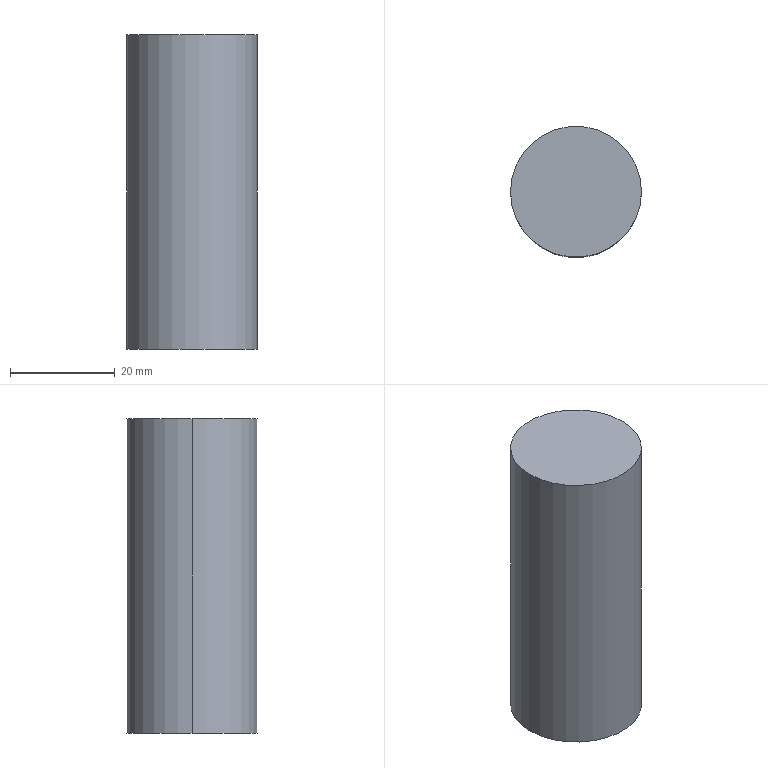Component | SolidWorks | Axis-1 | 1 solid | 4 faces | box 25 x 25 x 60 mm | volume 29452 mm3 | cylinder 2 | plane 2 | commonest cylinder face diameters 25 x2
build123d program:
from build123d import *

# Parameters (mm, degrees)
SKETCH1_R           = 12.5
BOSS_EXTRUDE1_DEPTH = 60


with BuildPart() as part:
    # Sketch1 → Boss-Extrude1 (new body)
    with BuildSketch(Plane.XY):
        Circle(SKETCH1_R)
    extrude(amount=BOSS_EXTRUDE1_DEPTH)


solid = part.part

# Placed as in the assembly
solid = solid.moved(Location((54.344, 1102.787, -13), (0, 0, 0)))
STEP:
#1=COLOUR_RGB('',0.7922,0.8196,0.9333);
#2=FILL_AREA_STYLE_COLOUR('',#1);
#3=FILL_AREA_STYLE('',(#2));
#4=SURFACE_STYLE_FILL_AREA(#3);
#5=SURFACE_SIDE_STYLE('',(#4));
#6=SURFACE_STYLE_USAGE(.BOTH.,#5);
#7=PRESENTATION_STYLE_ASSIGNMENT((#6));
#8=CARTESIAN_POINT('',(2.632,43.417,1.85));
#9=VERTEX_POINT('',#8);
#10=CARTESIAN_POINT('',(1.647,43.417,1.85));
#11=VERTEX_POINT('',#10);
#12=CARTESIAN_POINT('',(2.14,43.417,1.85));
#13=DIRECTION('',(0.,0.,1.));
#14=DIRECTION('',(1.,0.,0.));
#15=AXIS2_PLACEMENT_3D('',#12,#13,#14);
#16=CIRCLE('',#15,0.4921);
#17=EDGE_CURVE('',#9,#11,#16,.T.);
#18=ORIENTED_EDGE('',*,*,#17,.F.);
#19=CARTESIAN_POINT('',(2.632,43.417,-0.5118));
#20=VERTEX_POINT('',#19);
#21=CARTESIAN_POINT('',(2.632,43.417,1.85));
#22=DIRECTION('',(0.,0.,-1.));
#23=VECTOR('',#22,39.37);
#24=LINE('',#21,#23);
#25=EDGE_CURVE('',#9,#20,#24,.T.);
#26=ORIENTED_EDGE('',*,*,#25,.T.);
#27=CARTESIAN_POINT('',(1.647,43.417,-0.5118));
#28=VERTEX_POINT('',#27);
#29=CARTESIAN_POINT('',(2.14,43.417,-0.5118));
#30=DIRECTION('',(0.,0.,1.));
#31=DIRECTION('',(1.,0.,0.));
#32=AXIS2_PLACEMENT_3D('',#29,#30,#31);
#33=CIRCLE('',#32,0.4921);
#34=EDGE_CURVE('',#20,#28,#33,.T.);
#35=ORIENTED_EDGE('',*,*,#34,.T.);
#36=CARTESIAN_POINT('',(1.647,43.417,1.85));
#37=DIRECTION('',(0.,0.,-1.));
#38=VECTOR('',#37,39.37);
#39=LINE('',#36,#38);
#40=EDGE_CURVE('',#11,#28,#39,.T.);
#41=ORIENTED_EDGE('',*,*,#40,.F.);
#42=EDGE_LOOP('',(#18,#26,#35,#41));
#43=FACE_OUTER_BOUND('',#42,.T.);
#44=CARTESIAN_POINT('',(2.14,43.417,1.85));
#45=DIRECTION('',(0.,0.,-1.));
#46=DIRECTION('',(-1.,0.,0.));
#47=AXIS2_PLACEMENT_3D('',#44,#45,#46);
#48=CYLINDRICAL_SURFACE('',#47,0.4921);
#49=ADVANCED_FACE('',(#43),#48,.T.);
#50=ORIENTED_EDGE('',*,*,#25,.F.);
#51=CARTESIAN_POINT('',(2.14,43.417,1.85));
#52=DIRECTION('',(0.,0.,1.));
#53=DIRECTION('',(1.,0.,0.));
#54=AXIS2_PLACEMENT_3D('',#51,#52,#53);
#55=CIRCLE('',#54,0.4921);
#56=EDGE_CURVE('',#11,#9,#55,.T.);
#57=ORIENTED_EDGE('',*,*,#56,.F.);
#58=ORIENTED_EDGE('',*,*,#40,.T.);
#59=CARTESIAN_POINT('',(2.14,43.417,-0.5118));
#60=DIRECTION('',(0.,0.,1.));
#61=DIRECTION('',(1.,0.,0.));
#62=AXIS2_PLACEMENT_3D('',#59,#60,#61);
#63=CIRCLE('',#62,0.4921);
#64=EDGE_CURVE('',#28,#20,#63,.T.);
#65=ORIENTED_EDGE('',*,*,#64,.T.);
#66=EDGE_LOOP('',(#50,#57,#58,#65));
#67=FACE_OUTER_BOUND('',#66,.T.);
#68=CARTESIAN_POINT('',(2.14,43.417,1.85));
#69=DIRECTION('',(0.,0.,-1.));
#70=DIRECTION('',(-1.,0.,0.));
#71=AXIS2_PLACEMENT_3D('',#68,#69,#70);
#72=CYLINDRICAL_SURFACE('',#71,0.4921);
#73=ADVANCED_FACE('',(#67),#72,.T.);
#74=ORIENTED_EDGE('',*,*,#56,.T.);
#75=ORIENTED_EDGE('',*,*,#17,.T.);
#76=EDGE_LOOP('',(#74,#75));
#77=FACE_OUTER_BOUND('',#76,.T.);
#78=CARTESIAN_POINT('',(2.14,43.417,1.85));
#79=DIRECTION('',(0.,0.,1.));
#80=DIRECTION('',(1.,0.,0.));
#81=AXIS2_PLACEMENT_3D('',#78,#79,#80);
#82=PLANE('',#81);
#83=ADVANCED_FACE('',(#77),#82,.T.);
#84=ORIENTED_EDGE('',*,*,#64,.F.);
#85=ORIENTED_EDGE('',*,*,#34,.F.);
#86=EDGE_LOOP('',(#84,#85));
#87=FACE_OUTER_BOUND('',#86,.T.);
#88=CARTESIAN_POINT('',(2.14,43.417,-0.5118));
#89=DIRECTION('',(0.,0.,1.));
#90=DIRECTION('',(1.,0.,0.));
#91=AXIS2_PLACEMENT_3D('',#88,#89,#90);
#92=PLANE('',#91);
#93=ADVANCED_FACE('',(#87),#92,.F.);
#94=CLOSED_SHELL('',(#49,#73,#83,#93));
#95=MANIFOLD_SOLID_BREP('',#94);
#96=STYLED_ITEM('',(#7),#95);
#97=(LENGTH_UNIT()NAMED_UNIT(*)SI_UNIT($,.METRE.));
#98=LENGTH_MEASURE_WITH_UNIT(LENGTH_MEASURE(0.0254),#97);
#99=DIMENSIONAL_EXPONENTS(1.,0.,0.,0.,0.,0.,0.);
#100=(CONVERSION_BASED_UNIT('',#98)LENGTH_UNIT()NAMED_UNIT(#99));
#101=UNCERTAINTY_MEASURE_WITH_UNIT(LENGTH_MEASURE(0.00001),#100,'','');
#102=(NAMED_UNIT(*)PLANE_ANGLE_UNIT()SI_UNIT($,.RADIAN.));
#103=(NAMED_UNIT(*)SI_UNIT($,.STERADIAN.)SOLID_ANGLE_UNIT());
#104=(GEOMETRIC_REPRESENTATION_CONTEXT(3)GLOBAL_UNCERTAINTY_ASSIGNED_CONTEXT((#101))GLOBAL_UNIT_ASSIGNED_CONTEXT((#100,#102,#103))REPRESENTATION_CONTEXT('',''));
#105=MECHANICAL_DESIGN_GEOMETRIC_PRESENTATION_REPRESENTATION('',(#96),#104);
#106=PRESENTATION_LAYER_ASSIGNMENT('','',(#96));
#107=CARTESIAN_POINT('',(0.,0.,0.));
#108=DIRECTION('',(0.,0.,1.));
#109=DIRECTION('',(1.,0.,0.));
#110=AXIS2_PLACEMENT_3D('',#107,#108,#109);
#111=(LENGTH_UNIT()NAMED_UNIT(*)SI_UNIT($,.METRE.));
#112=LENGTH_MEASURE_WITH_UNIT(LENGTH_MEASURE(0.0254),#111);
#113=DIMENSIONAL_EXPONENTS(1.,0.,0.,0.,0.,0.,0.);
#114=(CONVERSION_BASED_UNIT('',#112)LENGTH_UNIT()NAMED_UNIT(#113));
#115=UNCERTAINTY_MEASURE_WITH_UNIT(LENGTH_MEASURE(0.00001),#114,'','');
#116=(NAMED_UNIT(*)PLANE_ANGLE_UNIT()SI_UNIT($,.RADIAN.));
#117=(NAMED_UNIT(*)SI_UNIT($,.STERADIAN.)SOLID_ANGLE_UNIT());
#118=(GEOMETRIC_REPRESENTATION_CONTEXT(3)GLOBAL_UNCERTAINTY_ASSIGNED_CONTEXT((#115))GLOBAL_UNIT_ASSIGNED_CONTEXT((#114,#116,#117))REPRESENTATION_CONTEXT('',''));
#119=ADVANCED_BREP_SHAPE_REPRESENTATION('',(#95,#110),#118);